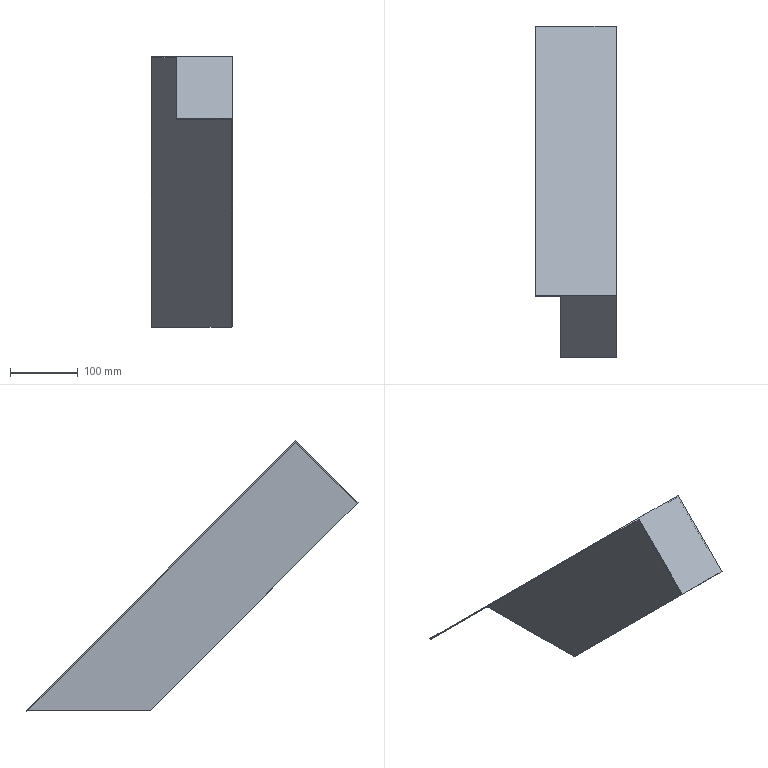Component | SolidWorks | RightSideBaffle-1 | 1 solid | 12 faces | box 120 x 491.44 x 400.93 mm | volume 284076 mm3 | plane 12
build123d program:
from build123d import *

# Parameters (mm, degrees)
EXTRUDE_THIN1_DEPTH = 565
CUT_EXTRUDE1_DEPTH  = 2
SKETCH3_W           = 83
SKETCH3_H           = 130
BOSS_EXTRUDE1_DEPTH = 2


with BuildPart() as part:
    # Sketch1 → Extrude-Thin1 (new body)
    with BuildSketch(Plane.XY):
        Polygon((-144.826, 24.07), (-24.826, 24.07), (-24.826, -105.93), (-26.826, -105.93), (-26.826, 22.07), (-144.826, 22.07), align=None)
    extrude(amount=EXTRUDE_THIN1_DEPTH)

    # Sketch2 → Cut-Extrude1 (cut)
    with BuildSketch(Plane(origin=(-24.826, 0, 0), x_dir=(0, 0, -1), z_dir=(1, 0, 0))):
        Polygon((0, 24.07), (-130, -105.93), (0, -105.93), align=None)
    extrude(amount=-CUT_EXTRUDE1_DEPTH, mode=Mode.SUBTRACT)

    # Sketch3 → Boss-Extrude1 (add)
    with BuildSketch(Plane.XY.offset(565)):
        with Locations((-66.326, -40.93)):
            Rectangle(SKETCH3_W, SKETCH3_H)
    extrude(amount=-BOSS_EXTRUDE1_DEPTH)


solid = part.part

# Placed as in the assembly
solid = solid.moved(Location((366.651, 211.717, -352.441), (45, 0, 0)))
STEP:
#1=CARTESIAN_POINT('',(13.379,-10.287,-1.151));
#2=VERTEX_POINT('',#1);
#3=CARTESIAN_POINT('',(13.379,1.767,-13.206));
#4=VERTEX_POINT('',#3);
#5=CARTESIAN_POINT('',(13.379,-10.343,-1.096));
#6=DIRECTION('',(0.,0.7071,-0.7071));
#7=VECTOR('',#6,39.37);
#8=LINE('',#5,#7);
#9=EDGE_CURVE('',#2,#4,#8,.T.);
#10=ORIENTED_EDGE('',*,*,#9,.F.);
#11=CARTESIAN_POINT('',(13.379,-6.724,2.412));
#12=VERTEX_POINT('',#11);
#13=CARTESIAN_POINT('',(13.379,-6.668,2.468));
#14=DIRECTION('',(-0.,0.7071,0.7071));
#15=VECTOR('',#14,39.37);
#16=LINE('',#13,#15);
#17=EDGE_CURVE('',#2,#12,#16,.T.);
#18=ORIENTED_EDGE('',*,*,#17,.T.);
#19=CARTESIAN_POINT('',(13.379,8.894,-13.206));
#20=VERTEX_POINT('',#19);
#21=CARTESIAN_POINT('',(13.379,-6.779,2.468));
#22=DIRECTION('',(0.,0.7071,-0.7071));
#23=VECTOR('',#22,39.37);
#24=LINE('',#21,#23);
#25=EDGE_CURVE('',#12,#20,#24,.T.);
#26=ORIENTED_EDGE('',*,*,#25,.T.);
#27=CARTESIAN_POINT('',(13.379,9.005,-13.206));
#28=DIRECTION('',(0.,-1.,-0.));
#29=VECTOR('',#28,39.37);
#30=LINE('',#27,#29);
#31=EDGE_CURVE('',#20,#4,#30,.T.);
#32=ORIENTED_EDGE('',*,*,#31,.T.);
#33=EDGE_LOOP('',(#10,#18,#26,#32));
#34=FACE_OUTER_BOUND('',#33,.T.);
#35=CARTESIAN_POINT('',(13.379,-6.724,2.523));
#36=DIRECTION('',(1.,0.,0.));
#37=DIRECTION('',(-0.,0.7071,0.7071));
#38=AXIS2_PLACEMENT_3D('',#35,#36,#37);
#39=PLANE('',#38);
#40=ADVANCED_FACE('',(#34),#39,.F.);
#41=CARTESIAN_POINT('',(13.458,1.767,-13.206));
#42=VERTEX_POINT('',#41);
#43=CARTESIAN_POINT('',(13.379,1.767,-13.206));
#44=DIRECTION('',(1.,0.,0.));
#45=VECTOR('',#44,39.37);
#46=LINE('',#43,#45);
#47=EDGE_CURVE('',#4,#42,#46,.T.);
#48=ORIENTED_EDGE('',*,*,#47,.T.);
#49=CARTESIAN_POINT('',(13.458,-10.343,-1.096));
#50=VERTEX_POINT('',#49);
#51=CARTESIAN_POINT('',(13.458,-10.343,-1.096));
#52=DIRECTION('',(0.,0.7071,-0.7071));
#53=VECTOR('',#52,39.37);
#54=LINE('',#51,#53);
#55=EDGE_CURVE('',#50,#42,#54,.T.);
#56=ORIENTED_EDGE('',*,*,#55,.F.);
#57=CARTESIAN_POINT('',(10.19,-10.343,-1.096));
#58=VERTEX_POINT('',#57);
#59=CARTESIAN_POINT('',(13.458,-10.343,-1.096));
#60=DIRECTION('',(-1.,0.,-0.));
#61=VECTOR('',#60,39.37);
#62=LINE('',#59,#61);
#63=EDGE_CURVE('',#50,#58,#62,.T.);
#64=ORIENTED_EDGE('',*,*,#63,.T.);
#65=CARTESIAN_POINT('',(10.19,-10.287,-1.151));
#66=VERTEX_POINT('',#65);
#67=CARTESIAN_POINT('',(10.19,-10.287,-1.151));
#68=DIRECTION('',(-0.,-0.7071,0.7071));
#69=VECTOR('',#68,39.37);
#70=LINE('',#67,#69);
#71=EDGE_CURVE('',#66,#58,#70,.T.);
#72=ORIENTED_EDGE('',*,*,#71,.F.);
#73=CARTESIAN_POINT('',(13.458,-10.287,-1.151));
#74=DIRECTION('',(1.,-0.,0.));
#75=VECTOR('',#74,39.37);
#76=LINE('',#73,#75);
#77=EDGE_CURVE('',#66,#2,#76,.T.);
#78=ORIENTED_EDGE('',*,*,#77,.T.);
#79=ORIENTED_EDGE('',*,*,#9,.T.);
#80=EDGE_LOOP('',(#48,#56,#64,#72,#78,#79));
#81=FACE_OUTER_BOUND('',#80,.T.);
#82=CARTESIAN_POINT('',(13.458,-10.343,-1.096));
#83=DIRECTION('',(0.,-0.7071,-0.7071));
#84=DIRECTION('',(0.,0.7071,-0.7071));
#85=AXIS2_PLACEMENT_3D('',#82,#83,#84);
#86=PLANE('',#85);
#87=ADVANCED_FACE('',(#81),#86,.T.);
#88=CARTESIAN_POINT('',(13.458,9.005,-13.206));
#89=VERTEX_POINT('',#88);
#90=CARTESIAN_POINT('',(13.458,9.005,-13.206));
#91=DIRECTION('',(0.,-1.,-0.));
#92=VECTOR('',#91,39.37);
#93=LINE('',#90,#92);
#94=EDGE_CURVE('',#89,#42,#93,.T.);
#95=ORIENTED_EDGE('',*,*,#94,.F.);
#96=CARTESIAN_POINT('',(13.458,-6.724,2.523));
#97=VERTEX_POINT('',#96);
#98=CARTESIAN_POINT('',(13.458,-6.724,2.523));
#99=DIRECTION('',(0.,0.7071,-0.7071));
#100=VECTOR('',#99,39.37);
#101=LINE('',#98,#100);
#102=EDGE_CURVE('',#97,#89,#101,.T.);
#103=ORIENTED_EDGE('',*,*,#102,.F.);
#104=CARTESIAN_POINT('',(13.458,-6.724,2.523));
#105=DIRECTION('',(0.,-0.7071,-0.7071));
#106=VECTOR('',#105,39.37);
#107=LINE('',#104,#106);
#108=EDGE_CURVE('',#97,#50,#107,.T.);
#109=ORIENTED_EDGE('',*,*,#108,.T.);
#110=ORIENTED_EDGE('',*,*,#55,.T.);
#111=EDGE_LOOP('',(#95,#103,#109,#110));
#112=FACE_OUTER_BOUND('',#111,.T.);
#113=CARTESIAN_POINT('',(13.458,-6.724,2.523));
#114=DIRECTION('',(1.,0.,0.));
#115=DIRECTION('',(-0.,0.7071,0.7071));
#116=AXIS2_PLACEMENT_3D('',#113,#114,#115);
#117=PLANE('',#116);
#118=ADVANCED_FACE('',(#112),#117,.T.);
#119=CARTESIAN_POINT('',(8.733,-6.724,2.523));
#120=VERTEX_POINT('',#119);
#121=CARTESIAN_POINT('',(8.733,-6.724,2.523));
#122=DIRECTION('',(1.,-0.,0.));
#123=VECTOR('',#122,39.37);
#124=LINE('',#121,#123);
#125=EDGE_CURVE('',#120,#97,#124,.T.);
#126=ORIENTED_EDGE('',*,*,#125,.T.);
#127=ORIENTED_EDGE('',*,*,#102,.T.);
#128=CARTESIAN_POINT('',(13.379,9.005,-13.206));
#129=VERTEX_POINT('',#128);
#130=CARTESIAN_POINT('',(13.379,9.005,-13.206));
#131=DIRECTION('',(1.,0.,0.));
#132=VECTOR('',#131,39.37);
#133=LINE('',#130,#132);
#134=EDGE_CURVE('',#129,#89,#133,.T.);
#135=ORIENTED_EDGE('',*,*,#134,.F.);
#136=CARTESIAN_POINT('',(8.733,9.005,-13.206));
#137=VERTEX_POINT('',#136);
#138=CARTESIAN_POINT('',(8.733,9.005,-13.206));
#139=DIRECTION('',(1.,-0.,0.));
#140=VECTOR('',#139,39.37);
#141=LINE('',#138,#140);
#142=EDGE_CURVE('',#137,#129,#141,.T.);
#143=ORIENTED_EDGE('',*,*,#142,.F.);
#144=CARTESIAN_POINT('',(8.733,-6.724,2.523));
#145=DIRECTION('',(0.,0.7071,-0.7071));
#146=VECTOR('',#145,39.37);
#147=LINE('',#144,#146);
#148=EDGE_CURVE('',#120,#137,#147,.T.);
#149=ORIENTED_EDGE('',*,*,#148,.F.);
#150=EDGE_LOOP('',(#126,#127,#135,#143,#149));
#151=FACE_OUTER_BOUND('',#150,.T.);
#152=CARTESIAN_POINT('',(8.733,-6.724,2.523));
#153=DIRECTION('',(-0.,0.7071,0.7071));
#154=DIRECTION('',(-0.,-0.7071,0.7071));
#155=AXIS2_PLACEMENT_3D('',#152,#153,#154);
#156=PLANE('',#155);
#157=ADVANCED_FACE('',(#151),#156,.T.);
#158=CARTESIAN_POINT('',(8.733,8.95,-13.261));
#159=VERTEX_POINT('',#158);
#160=CARTESIAN_POINT('',(8.733,8.95,-13.261));
#161=DIRECTION('',(-0.,0.7071,0.7071));
#162=VECTOR('',#161,39.37);
#163=LINE('',#160,#162);
#164=EDGE_CURVE('',#159,#137,#163,.T.);
#165=ORIENTED_EDGE('',*,*,#164,.F.);
#166=CARTESIAN_POINT('',(8.733,-6.779,2.468));
#167=VERTEX_POINT('',#166);
#168=CARTESIAN_POINT('',(8.733,-6.779,2.468));
#169=DIRECTION('',(0.,0.7071,-0.7071));
#170=VECTOR('',#169,39.37);
#171=LINE('',#168,#170);
#172=EDGE_CURVE('',#167,#159,#171,.T.);
#173=ORIENTED_EDGE('',*,*,#172,.F.);
#174=CARTESIAN_POINT('',(8.733,-6.779,2.468));
#175=DIRECTION('',(-0.,0.7071,0.7071));
#176=VECTOR('',#175,39.37);
#177=LINE('',#174,#176);
#178=EDGE_CURVE('',#167,#120,#177,.T.);
#179=ORIENTED_EDGE('',*,*,#178,.T.);
#180=ORIENTED_EDGE('',*,*,#148,.T.);
#181=EDGE_LOOP('',(#165,#173,#179,#180));
#182=FACE_OUTER_BOUND('',#181,.T.);
#183=CARTESIAN_POINT('',(8.733,-6.779,2.468));
#184=DIRECTION('',(-1.,0.,-0.));
#185=DIRECTION('',(-0.,-0.7071,0.7071));
#186=AXIS2_PLACEMENT_3D('',#183,#184,#185);
#187=PLANE('',#186);
#188=ADVANCED_FACE('',(#182),#187,.T.);
#189=CARTESIAN_POINT('',(10.19,-6.724,2.412));
#190=VERTEX_POINT('',#189);
#191=CARTESIAN_POINT('',(8.733,-6.724,2.412));
#192=DIRECTION('',(-1.,0.,-0.));
#193=VECTOR('',#192,39.37);
#194=LINE('',#191,#193);
#195=EDGE_CURVE('',#12,#190,#194,.T.);
#196=ORIENTED_EDGE('',*,*,#195,.T.);
#197=CARTESIAN_POINT('',(10.19,-6.779,2.468));
#198=VERTEX_POINT('',#197);
#199=CARTESIAN_POINT('',(10.19,-6.779,2.468));
#200=DIRECTION('',(-0.,-0.7071,0.7071));
#201=VECTOR('',#200,39.37);
#202=LINE('',#199,#201);
#203=EDGE_CURVE('',#190,#198,#202,.T.);
#204=ORIENTED_EDGE('',*,*,#203,.T.);
#205=CARTESIAN_POINT('',(8.733,-6.779,2.468));
#206=DIRECTION('',(1.,-0.,0.));
#207=VECTOR('',#206,39.37);
#208=LINE('',#205,#207);
#209=EDGE_CURVE('',#167,#198,#208,.T.);
#210=ORIENTED_EDGE('',*,*,#209,.F.);
#211=ORIENTED_EDGE('',*,*,#172,.T.);
#212=CARTESIAN_POINT('',(13.379,8.95,-13.261));
#213=VERTEX_POINT('',#212);
#214=CARTESIAN_POINT('',(8.733,8.95,-13.261));
#215=DIRECTION('',(1.,-0.,0.));
#216=VECTOR('',#215,39.37);
#217=LINE('',#214,#216);
#218=EDGE_CURVE('',#159,#213,#217,.T.);
#219=ORIENTED_EDGE('',*,*,#218,.T.);
#220=CARTESIAN_POINT('',(13.379,-6.779,2.468));
#221=DIRECTION('',(-0.,-0.7071,0.7071));
#222=VECTOR('',#221,39.37);
#223=LINE('',#220,#222);
#224=EDGE_CURVE('',#213,#20,#223,.T.);
#225=ORIENTED_EDGE('',*,*,#224,.T.);
#226=ORIENTED_EDGE('',*,*,#25,.F.);
#227=EDGE_LOOP('',(#196,#204,#210,#211,#219,#225,#226));
#228=FACE_OUTER_BOUND('',#227,.T.);
#229=CARTESIAN_POINT('',(8.733,-6.779,2.468));
#230=DIRECTION('',(-0.,0.7071,0.7071));
#231=DIRECTION('',(-0.,-0.7071,0.7071));
#232=AXIS2_PLACEMENT_3D('',#229,#230,#231);
#233=PLANE('',#232);
#234=ADVANCED_FACE('',(#228),#233,.F.);
#235=CARTESIAN_POINT('',(10.19,-6.724,2.523));
#236=DIRECTION('',(0.,-0.7071,-0.7071));
#237=VECTOR('',#236,39.37);
#238=LINE('',#235,#237);
#239=EDGE_CURVE('',#198,#58,#238,.T.);
#240=ORIENTED_EDGE('',*,*,#239,.T.);
#241=ORIENTED_EDGE('',*,*,#63,.F.);
#242=ORIENTED_EDGE('',*,*,#108,.F.);
#243=ORIENTED_EDGE('',*,*,#125,.F.);
#244=ORIENTED_EDGE('',*,*,#178,.F.);
#245=ORIENTED_EDGE('',*,*,#209,.T.);
#246=EDGE_LOOP('',(#240,#241,#242,#243,#244,#245));
#247=FACE_OUTER_BOUND('',#246,.T.);
#248=CARTESIAN_POINT('',(14.435,-7.394,1.853));
#249=DIRECTION('',(0.,0.7071,-0.7071));
#250=DIRECTION('',(-1.,0.,-0.));
#251=AXIS2_PLACEMENT_3D('',#248,#249,#250);
#252=PLANE('',#251);
#253=ADVANCED_FACE('',(#247),#252,.F.);
#254=CARTESIAN_POINT('',(13.379,8.335,-13.876));
#255=DIRECTION('',(-0.,0.7071,0.7071));
#256=VECTOR('',#255,39.37);
#257=LINE('',#254,#256);
#258=EDGE_CURVE('',#213,#129,#257,.T.);
#259=ORIENTED_EDGE('',*,*,#258,.F.);
#260=ORIENTED_EDGE('',*,*,#218,.F.);
#261=ORIENTED_EDGE('',*,*,#164,.T.);
#262=ORIENTED_EDGE('',*,*,#142,.T.);
#263=EDGE_LOOP('',(#259,#260,#261,#262));
#264=FACE_OUTER_BOUND('',#263,.T.);
#265=CARTESIAN_POINT('',(14.435,8.335,-13.876));
#266=DIRECTION('',(0.,0.7071,-0.7071));
#267=DIRECTION('',(-1.,0.,-0.));
#268=AXIS2_PLACEMENT_3D('',#265,#266,#267);
#269=PLANE('',#268);
#270=ADVANCED_FACE('',(#264),#269,.T.);
#271=ORIENTED_EDGE('',*,*,#258,.T.);
#272=CARTESIAN_POINT('',(13.379,9.005,-13.206));
#273=DIRECTION('',(0.,-1.,-0.));
#274=VECTOR('',#273,39.37);
#275=LINE('',#272,#274);
#276=EDGE_CURVE('',#129,#20,#275,.T.);
#277=ORIENTED_EDGE('',*,*,#276,.T.);
#278=ORIENTED_EDGE('',*,*,#224,.F.);
#279=EDGE_LOOP('',(#271,#277,#278));
#280=FACE_OUTER_BOUND('',#279,.T.);
#281=CARTESIAN_POINT('',(13.379,8.335,-13.876));
#282=DIRECTION('',(-1.,-0.,-0.));
#283=DIRECTION('',(0.,-0.7071,-0.7071));
#284=AXIS2_PLACEMENT_3D('',#281,#282,#283);
#285=PLANE('',#284);
#286=ADVANCED_FACE('',(#280),#285,.F.);
#287=ORIENTED_EDGE('',*,*,#94,.T.);
#288=ORIENTED_EDGE('',*,*,#47,.F.);
#289=ORIENTED_EDGE('',*,*,#31,.F.);
#290=ORIENTED_EDGE('',*,*,#276,.F.);
#291=ORIENTED_EDGE('',*,*,#134,.T.);
#292=EDGE_LOOP('',(#287,#288,#289,#290,#291));
#293=FACE_OUTER_BOUND('',#292,.T.);
#294=CARTESIAN_POINT('',(13.379,9.005,-13.206));
#295=DIRECTION('',(-0.,-0.,1.));
#296=DIRECTION('',(-0.,-1.,-0.));
#297=AXIS2_PLACEMENT_3D('',#294,#295,#296);
#298=PLANE('',#297);
#299=ADVANCED_FACE('',(#293),#298,.F.);
#300=ORIENTED_EDGE('',*,*,#17,.F.);
#301=ORIENTED_EDGE('',*,*,#77,.F.);
#302=CARTESIAN_POINT('',(10.19,-6.668,2.468));
#303=DIRECTION('',(0.,-0.7071,-0.7071));
#304=VECTOR('',#303,39.37);
#305=LINE('',#302,#304);
#306=EDGE_CURVE('',#190,#66,#305,.T.);
#307=ORIENTED_EDGE('',*,*,#306,.F.);
#308=ORIENTED_EDGE('',*,*,#195,.F.);
#309=EDGE_LOOP('',(#300,#301,#307,#308));
#310=FACE_OUTER_BOUND('',#309,.T.);
#311=CARTESIAN_POINT('',(14.435,-7.338,1.798));
#312=DIRECTION('',(0.,0.7071,-0.7071));
#313=DIRECTION('',(-1.,0.,-0.));
#314=AXIS2_PLACEMENT_3D('',#311,#312,#313);
#315=PLANE('',#314);
#316=ADVANCED_FACE('',(#310),#315,.T.);
#317=ORIENTED_EDGE('',*,*,#203,.F.);
#318=ORIENTED_EDGE('',*,*,#306,.T.);
#319=ORIENTED_EDGE('',*,*,#71,.T.);
#320=ORIENTED_EDGE('',*,*,#239,.F.);
#321=EDGE_LOOP('',(#317,#318,#319,#320));
#322=FACE_OUTER_BOUND('',#321,.T.);
#323=CARTESIAN_POINT('',(10.19,-6.668,2.468));
#324=DIRECTION('',(-1.,0.,-0.));
#325=DIRECTION('',(-0.,-0.7071,0.7071));
#326=AXIS2_PLACEMENT_3D('',#323,#324,#325);
#327=PLANE('',#326);
#328=ADVANCED_FACE('',(#322),#327,.T.);
#329=CLOSED_SHELL('',(#40,#87,#118,#157,#188,#234,#253,#270,#286,#299,#316,#328));
#330=MANIFOLD_SOLID_BREP('',#329);
#331=CARTESIAN_POINT('',(0.,0.,0.));
#332=DIRECTION('',(0.,0.,1.));
#333=DIRECTION('',(1.,0.,0.));
#334=AXIS2_PLACEMENT_3D('',#331,#332,#333);
#335=(LENGTH_UNIT()NAMED_UNIT(*)SI_UNIT($,.METRE.));
#336=LENGTH_MEASURE_WITH_UNIT(LENGTH_MEASURE(0.0254),#335);
#337=DIMENSIONAL_EXPONENTS(1.,0.,0.,0.,0.,0.,0.);
#338=(CONVERSION_BASED_UNIT('',#336)LENGTH_UNIT()NAMED_UNIT(#337));
#339=UNCERTAINTY_MEASURE_WITH_UNIT(LENGTH_MEASURE(0.00001),#338,'','');
#340=(NAMED_UNIT(*)PLANE_ANGLE_UNIT()SI_UNIT($,.RADIAN.));
#341=(NAMED_UNIT(*)SI_UNIT($,.STERADIAN.)SOLID_ANGLE_UNIT());
#342=(GEOMETRIC_REPRESENTATION_CONTEXT(3)GLOBAL_UNCERTAINTY_ASSIGNED_CONTEXT((#339))GLOBAL_UNIT_ASSIGNED_CONTEXT((#338,#340,#341))REPRESENTATION_CONTEXT('',''));
#343=ADVANCED_BREP_SHAPE_REPRESENTATION('',(#330,#334),#342);
#344=COLOUR_RGB('',0.7922,0.8196,0.9333);
#345=FILL_AREA_STYLE_COLOUR('',#344);
#346=FILL_AREA_STYLE('',(#345));
#347=SURFACE_STYLE_FILL_AREA(#346);
#348=SURFACE_SIDE_STYLE('',(#347));
#349=SURFACE_STYLE_USAGE(.BOTH.,#348);
#350=PRESENTATION_STYLE_ASSIGNMENT((#349));
#351=STYLED_ITEM('',(#350),#330);
#352=PRESENTATION_LAYER_ASSIGNMENT('','',(#351));
#353=(LENGTH_UNIT()NAMED_UNIT(*)SI_UNIT($,.METRE.));
#354=LENGTH_MEASURE_WITH_UNIT(LENGTH_MEASURE(0.0254),#353);
#355=DIMENSIONAL_EXPONENTS(1.,0.,0.,0.,0.,0.,0.);
#356=(CONVERSION_BASED_UNIT('',#354)LENGTH_UNIT()NAMED_UNIT(#355));
#357=UNCERTAINTY_MEASURE_WITH_UNIT(LENGTH_MEASURE(0.00001),#356,'','');
#358=(NAMED_UNIT(*)PLANE_ANGLE_UNIT()SI_UNIT($,.RADIAN.));
#359=(NAMED_UNIT(*)SI_UNIT($,.STERADIAN.)SOLID_ANGLE_UNIT());
#360=(GEOMETRIC_REPRESENTATION_CONTEXT(3)GLOBAL_UNCERTAINTY_ASSIGNED_CONTEXT((#357))GLOBAL_UNIT_ASSIGNED_CONTEXT((#356,#358,#359))REPRESENTATION_CONTEXT('',''));
#361=MECHANICAL_DESIGN_GEOMETRIC_PRESENTATION_REPRESENTATION('',(#351),#360);